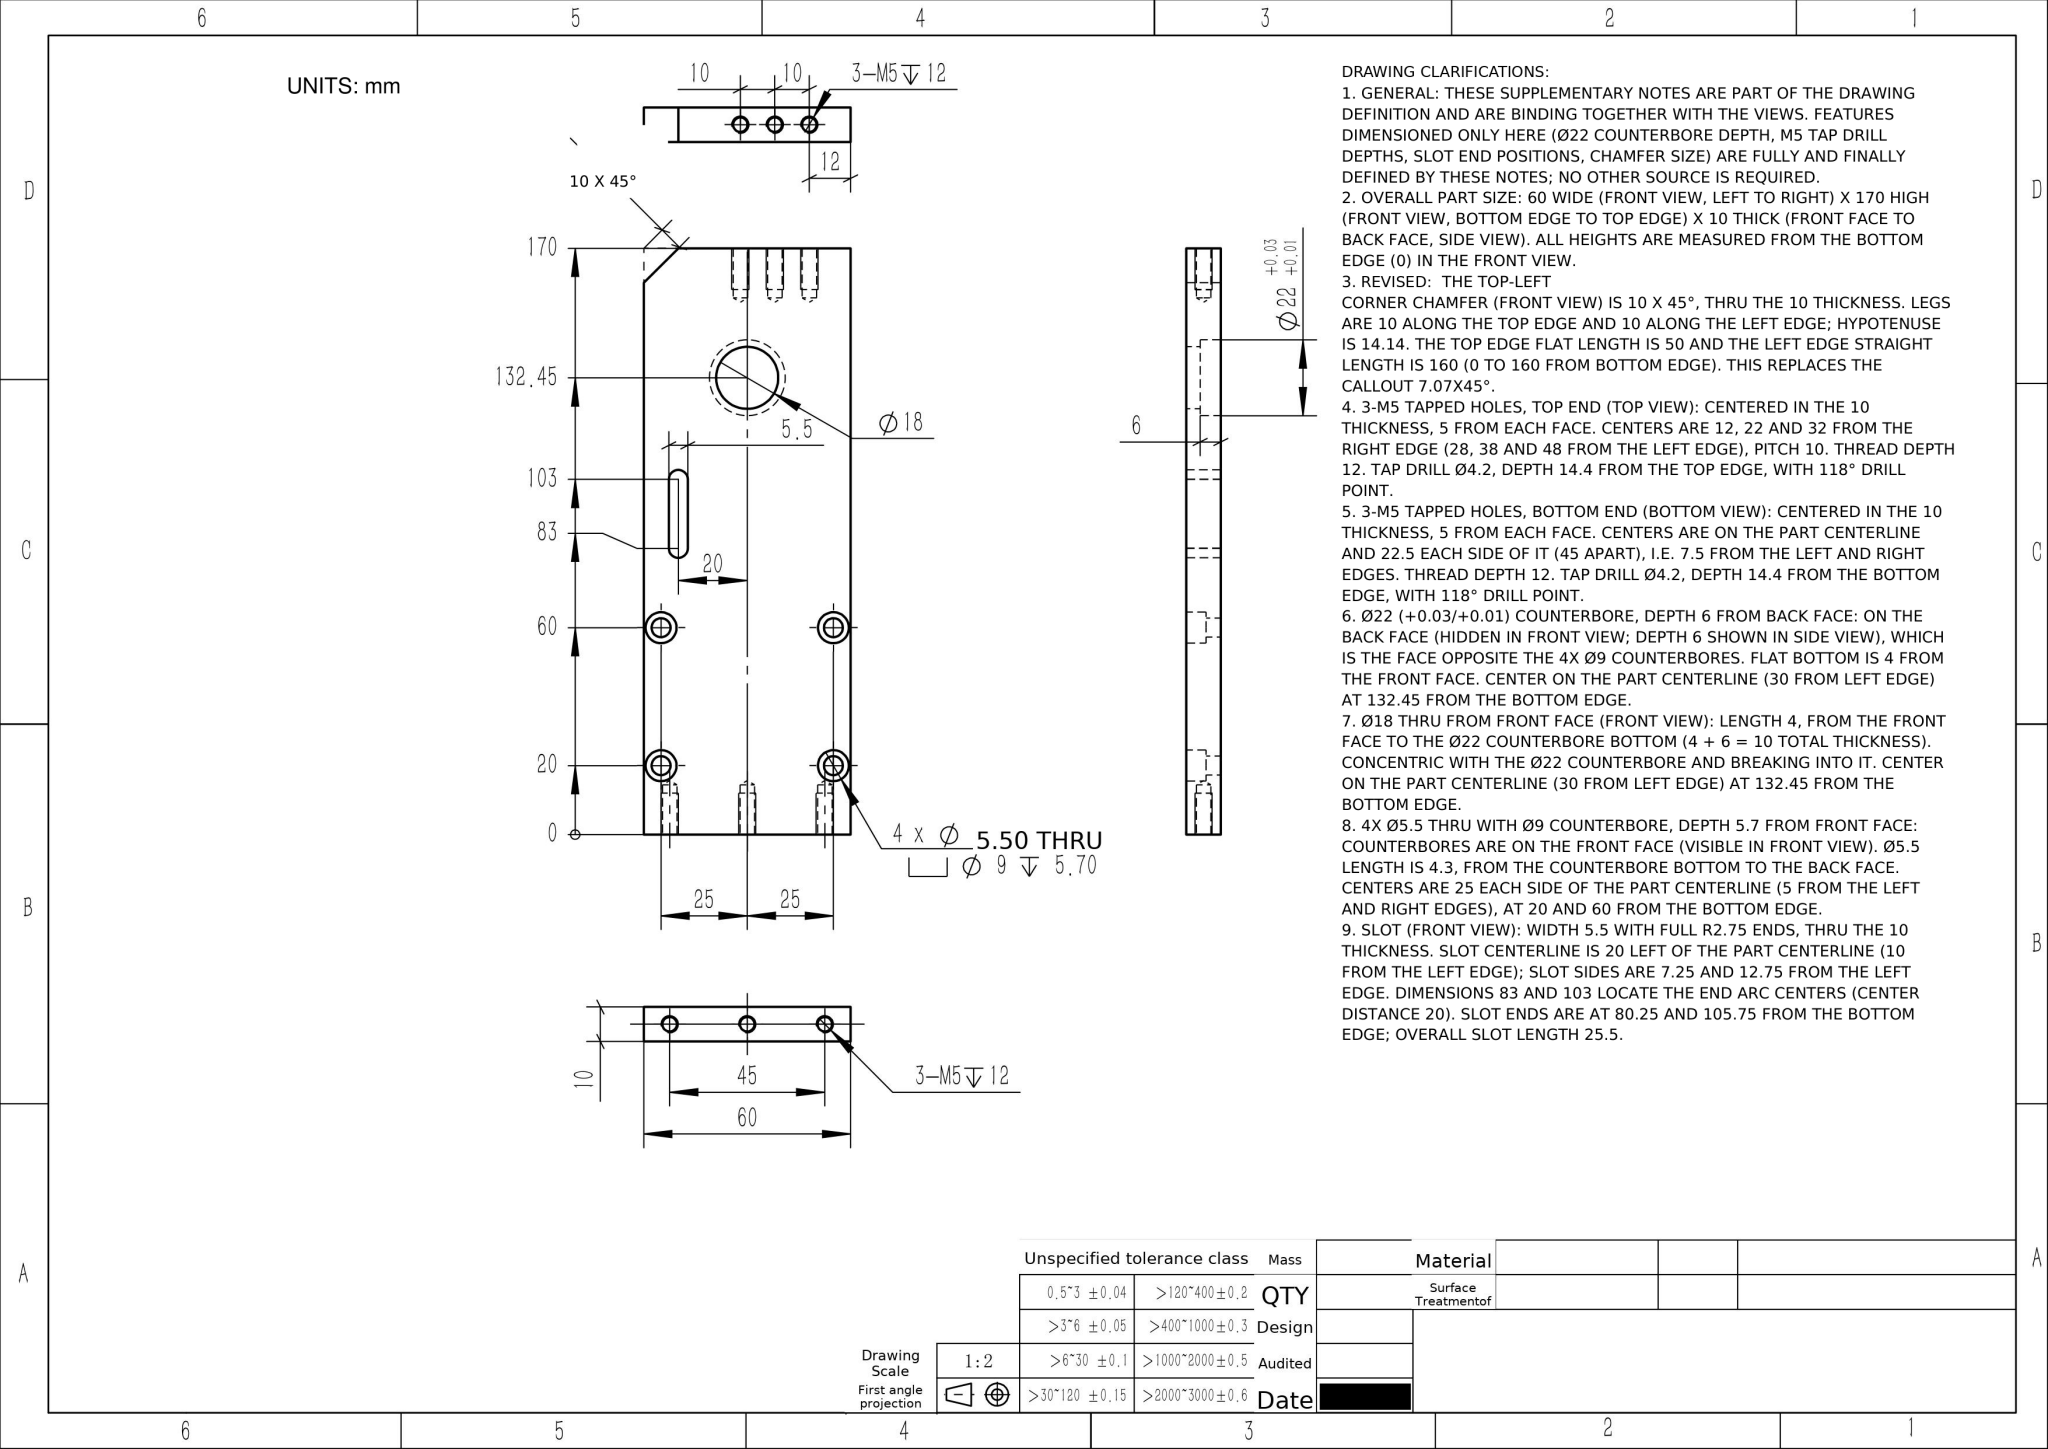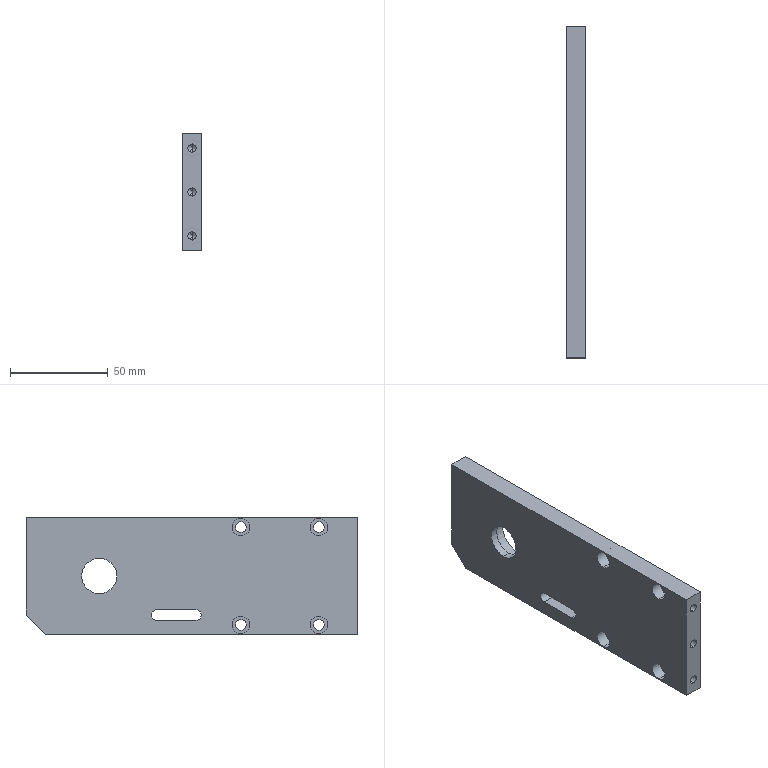Part | NX | mm | 1 solid | 60 faces | box 10 x 170 x 60 mm | volume 93773 mm3 | cylinder 34 | plane 14 | cone 12 | commonest cylinder face diameters 4.2 x12 5.5 x10 9 x8 18 x2 22 x2